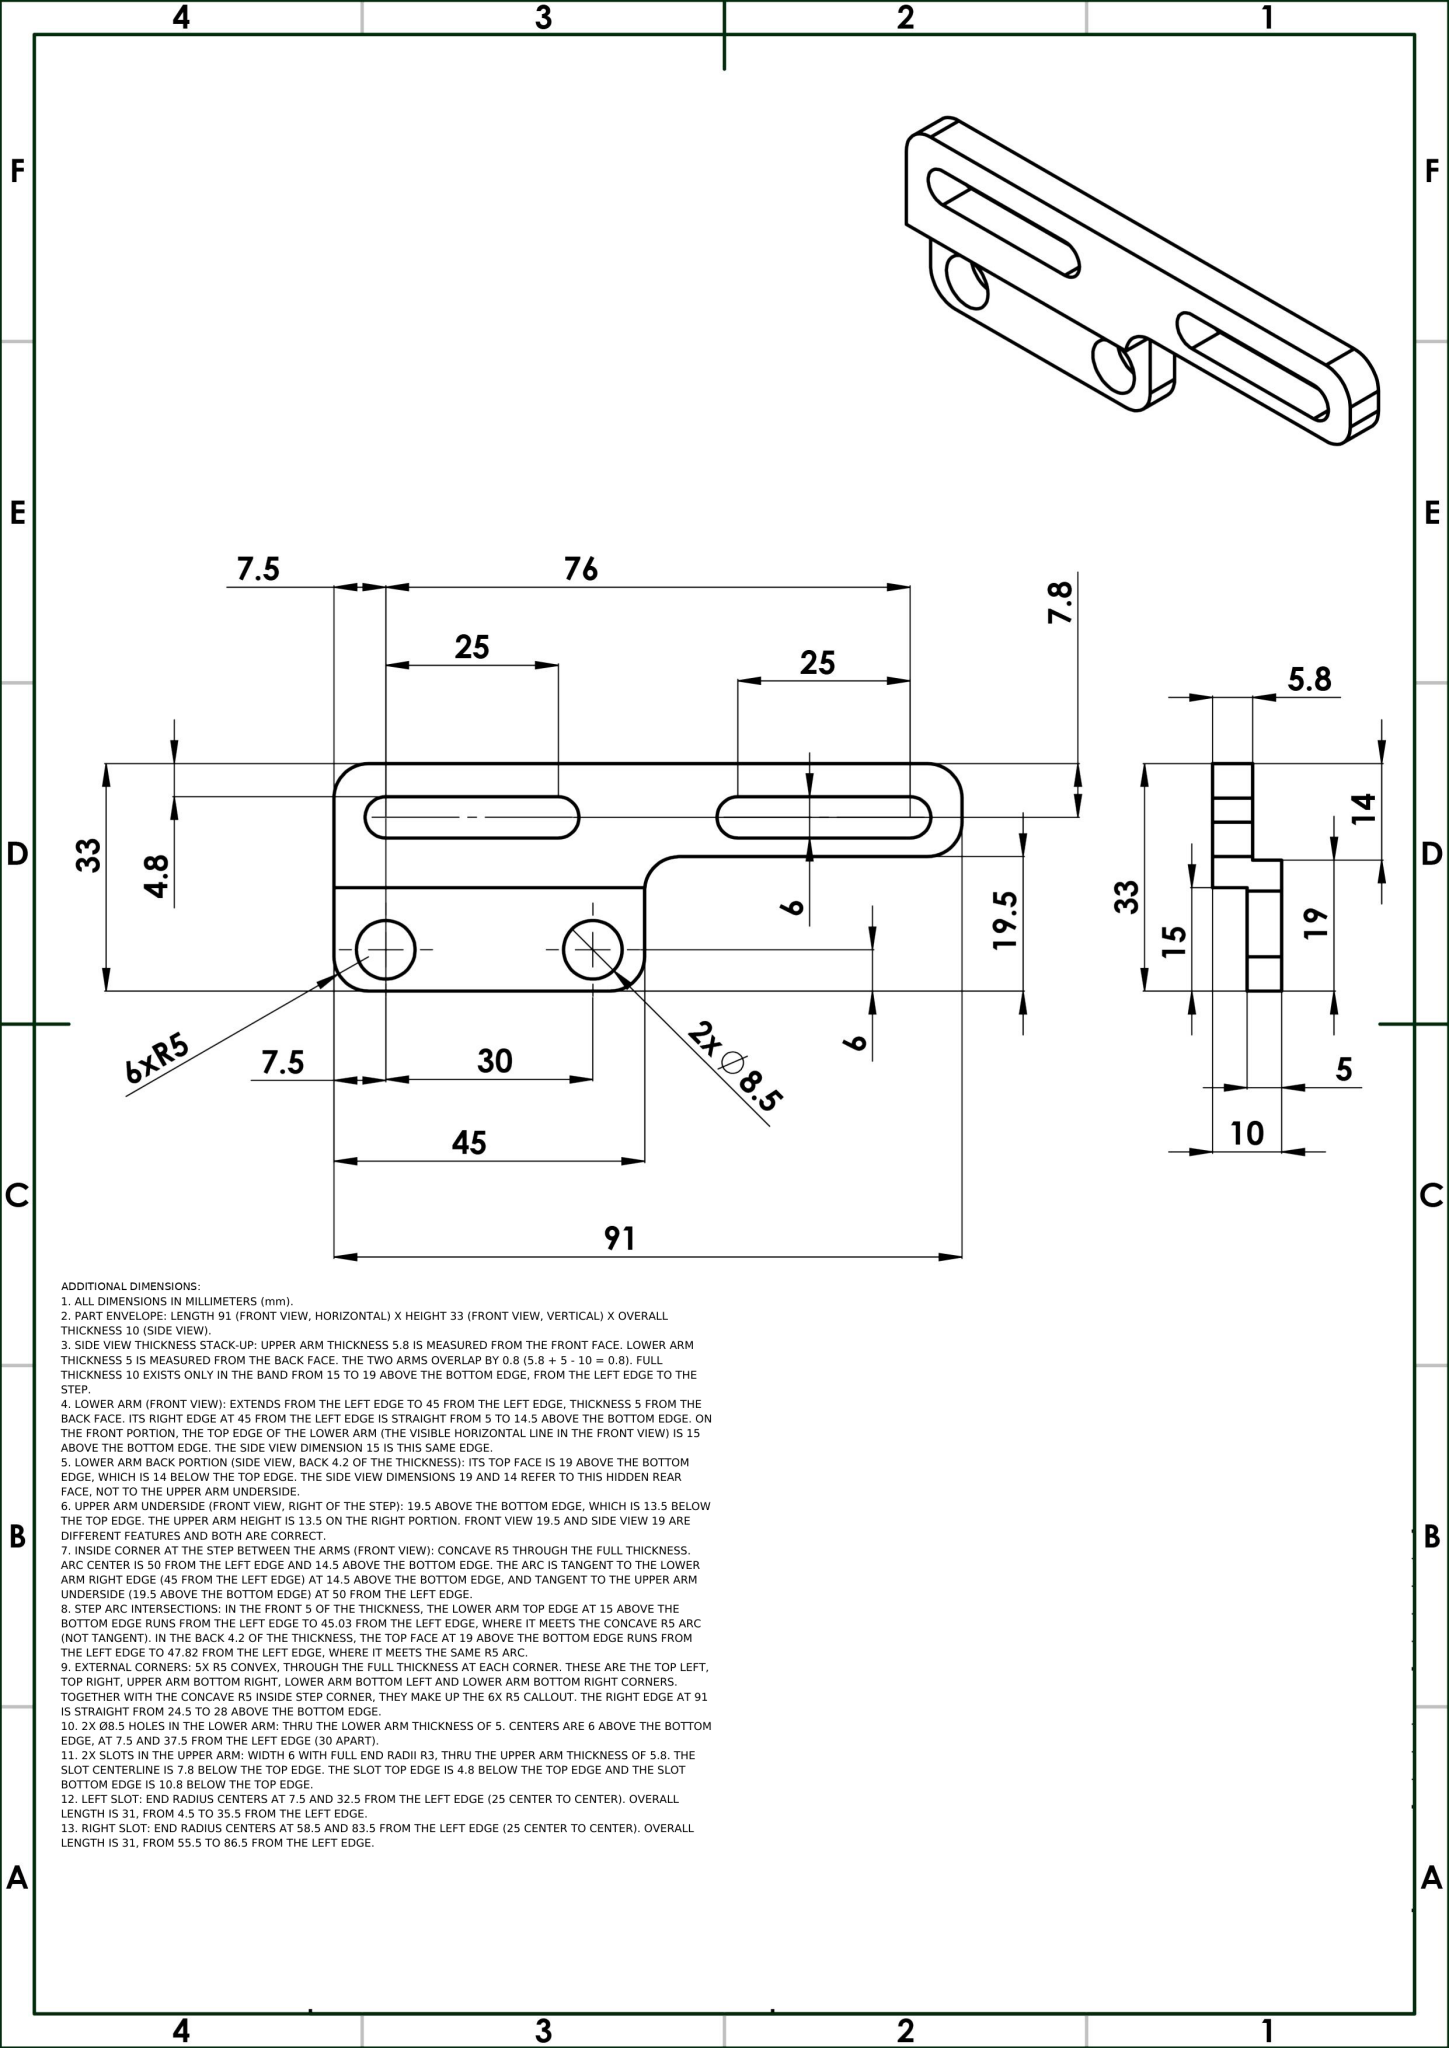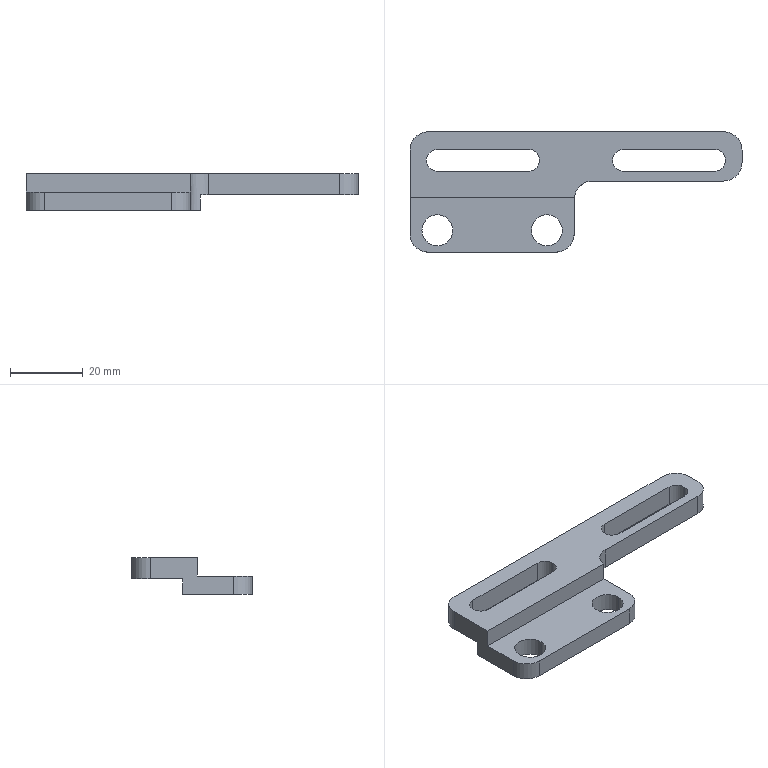Part | NX | mm | 1 solid | 32 faces | box 91 x 33 x 10 mm | volume 9695 mm3 | cylinder 16 | plane 16 | commonest cylinder face diameters 6 x6 10 x6 8.5 x4
STEP:
#1=CARTESIAN_POINT('',(11.75,-9.,0.));
#2=VERTEX_POINT('',#1);
#3=CARTESIAN_POINT('',(3.25,-9.,0.));
#4=VERTEX_POINT('',#3);
#5=CARTESIAN_POINT('',(7.5,-9.,0.));
#6=DIRECTION('',(0.,0.,-1.));
#7=DIRECTION('',(-1.,0.,0.));
#8=AXIS2_PLACEMENT_3D('',#5,#6,#7);
#9=CIRCLE('',#8,4.25);
#10=EDGE_CURVE('',#2,#4,#9,.T.);
#11=ORIENTED_EDGE('',*,*,#10,.F.);
#12=CARTESIAN_POINT('',(11.75,-9.,-5.));
#13=VERTEX_POINT('',#12);
#14=CARTESIAN_POINT('',(11.75,-9.,20.));
#15=DIRECTION('',(0.,0.,-1.));
#16=VECTOR('',#15,1000.);
#17=LINE('',#14,#16);
#18=EDGE_CURVE('',#2,#13,#17,.T.);
#19=ORIENTED_EDGE('',*,*,#18,.T.);
#20=CARTESIAN_POINT('',(3.25,-9.,-5.));
#21=VERTEX_POINT('',#20);
#22=CARTESIAN_POINT('',(7.5,-9.,-5.));
#23=DIRECTION('',(0.,0.,-1.));
#24=DIRECTION('',(-1.,0.,0.));
#25=AXIS2_PLACEMENT_3D('',#22,#23,#24);
#26=CIRCLE('',#25,4.25);
#27=EDGE_CURVE('',#13,#21,#26,.T.);
#28=ORIENTED_EDGE('',*,*,#27,.T.);
#29=CARTESIAN_POINT('',(3.25,-9.,20.));
#30=DIRECTION('',(0.,0.,-1.));
#31=VECTOR('',#30,1000.);
#32=LINE('',#29,#31);
#33=EDGE_CURVE('',#4,#21,#32,.T.);
#34=ORIENTED_EDGE('',*,*,#33,.F.);
#35=EDGE_LOOP('',(#11,#19,#28,#34));
#36=FACE_OUTER_BOUND('',#35,.T.);
#37=CARTESIAN_POINT('',(7.5,-9.,20.));
#38=DIRECTION('',(0.,0.,-1.));
#39=DIRECTION('',(-1.,0.,0.));
#40=AXIS2_PLACEMENT_3D('',#37,#38,#39);
#41=CYLINDRICAL_SURFACE('',#40,4.25);
#42=ADVANCED_FACE('',(#36),#41,.F.);
#43=CARTESIAN_POINT('',(41.75,-9.,0.));
#44=VERTEX_POINT('',#43);
#45=CARTESIAN_POINT('',(33.25,-9.,0.));
#46=VERTEX_POINT('',#45);
#47=CARTESIAN_POINT('',(37.5,-9.,0.));
#48=DIRECTION('',(0.,0.,-1.));
#49=DIRECTION('',(-1.,0.,0.));
#50=AXIS2_PLACEMENT_3D('',#47,#48,#49);
#51=CIRCLE('',#50,4.25);
#52=EDGE_CURVE('',#44,#46,#51,.T.);
#53=ORIENTED_EDGE('',*,*,#52,.F.);
#54=CARTESIAN_POINT('',(41.75,-9.,-5.));
#55=VERTEX_POINT('',#54);
#56=CARTESIAN_POINT('',(41.75,-9.,20.));
#57=DIRECTION('',(0.,0.,-1.));
#58=VECTOR('',#57,1000.);
#59=LINE('',#56,#58);
#60=EDGE_CURVE('',#44,#55,#59,.T.);
#61=ORIENTED_EDGE('',*,*,#60,.T.);
#62=CARTESIAN_POINT('',(33.25,-9.,-5.));
#63=VERTEX_POINT('',#62);
#64=CARTESIAN_POINT('',(37.5,-9.,-5.));
#65=DIRECTION('',(0.,0.,-1.));
#66=DIRECTION('',(-1.,0.,0.));
#67=AXIS2_PLACEMENT_3D('',#64,#65,#66);
#68=CIRCLE('',#67,4.25);
#69=EDGE_CURVE('',#55,#63,#68,.T.);
#70=ORIENTED_EDGE('',*,*,#69,.T.);
#71=CARTESIAN_POINT('',(33.25,-9.,20.));
#72=DIRECTION('',(0.,0.,-1.));
#73=VECTOR('',#72,1000.);
#74=LINE('',#71,#73);
#75=EDGE_CURVE('',#46,#63,#74,.T.);
#76=ORIENTED_EDGE('',*,*,#75,.F.);
#77=EDGE_LOOP('',(#53,#61,#70,#76));
#78=FACE_OUTER_BOUND('',#77,.T.);
#79=CARTESIAN_POINT('',(37.5,-9.,20.));
#80=DIRECTION('',(0.,0.,-1.));
#81=DIRECTION('',(-1.,0.,0.));
#82=AXIS2_PLACEMENT_3D('',#79,#80,#81);
#83=CYLINDRICAL_SURFACE('',#82,4.25);
#84=ADVANCED_FACE('',(#78),#83,.F.);
#85=CARTESIAN_POINT('',(83.5,13.2,-0.8));
#86=VERTEX_POINT('',#85);
#87=CARTESIAN_POINT('',(86.5,10.2,-0.8));
#88=VERTEX_POINT('',#87);
#89=CARTESIAN_POINT('',(83.5,10.2,-0.8));
#90=DIRECTION('',(0.,0.,-1.));
#91=DIRECTION('',(-1.,0.,0.));
#92=AXIS2_PLACEMENT_3D('',#89,#90,#91);
#93=CIRCLE('',#92,3.);
#94=EDGE_CURVE('',#86,#88,#93,.T.);
#95=ORIENTED_EDGE('',*,*,#94,.T.);
#96=CARTESIAN_POINT('',(86.5,10.2,5.));
#97=VERTEX_POINT('',#96);
#98=CARTESIAN_POINT('',(86.5,10.2,-5.));
#99=DIRECTION('',(0.,0.,1.));
#100=VECTOR('',#99,1000.);
#101=LINE('',#98,#100);
#102=EDGE_CURVE('',#88,#97,#101,.T.);
#103=ORIENTED_EDGE('',*,*,#102,.T.);
#104=CARTESIAN_POINT('',(83.5,13.2,5.));
#105=VERTEX_POINT('',#104);
#106=CARTESIAN_POINT('',(83.5,10.2,5.));
#107=DIRECTION('',(0.,0.,1.));
#108=DIRECTION('',(1.,0.,0.));
#109=AXIS2_PLACEMENT_3D('',#106,#107,#108);
#110=CIRCLE('',#109,3.);
#111=EDGE_CURVE('',#97,#105,#110,.T.);
#112=ORIENTED_EDGE('',*,*,#111,.T.);
#113=CARTESIAN_POINT('',(83.5,13.2,-5.));
#114=DIRECTION('',(0.,0.,1.));
#115=VECTOR('',#114,1000.);
#116=LINE('',#113,#115);
#117=EDGE_CURVE('',#86,#105,#116,.T.);
#118=ORIENTED_EDGE('',*,*,#117,.F.);
#119=EDGE_LOOP('',(#95,#103,#112,#118));
#120=FACE_OUTER_BOUND('',#119,.T.);
#121=CARTESIAN_POINT('',(83.5,10.2,-5.));
#122=DIRECTION('',(0.,0.,1.));
#123=DIRECTION('',(1.,0.,0.));
#124=AXIS2_PLACEMENT_3D('',#121,#122,#123);
#125=CYLINDRICAL_SURFACE('',#124,3.);
#126=ADVANCED_FACE('',(#120),#125,.F.);
#127=CARTESIAN_POINT('',(32.5,13.2,-0.8));
#128=VERTEX_POINT('',#127);
#129=CARTESIAN_POINT('',(35.5,10.2,-0.8));
#130=VERTEX_POINT('',#129);
#131=CARTESIAN_POINT('',(32.5,10.2,-0.8));
#132=DIRECTION('',(0.,0.,-1.));
#133=DIRECTION('',(-1.,0.,0.));
#134=AXIS2_PLACEMENT_3D('',#131,#132,#133);
#135=CIRCLE('',#134,3.);
#136=EDGE_CURVE('',#128,#130,#135,.T.);
#137=ORIENTED_EDGE('',*,*,#136,.T.);
#138=CARTESIAN_POINT('',(35.5,10.2,5.));
#139=VERTEX_POINT('',#138);
#140=CARTESIAN_POINT('',(35.5,10.2,-5.));
#141=DIRECTION('',(0.,0.,1.));
#142=VECTOR('',#141,1000.);
#143=LINE('',#140,#142);
#144=EDGE_CURVE('',#130,#139,#143,.T.);
#145=ORIENTED_EDGE('',*,*,#144,.T.);
#146=CARTESIAN_POINT('',(32.5,13.2,5.));
#147=VERTEX_POINT('',#146);
#148=CARTESIAN_POINT('',(32.5,10.2,5.));
#149=DIRECTION('',(0.,0.,1.));
#150=DIRECTION('',(1.,0.,0.));
#151=AXIS2_PLACEMENT_3D('',#148,#149,#150);
#152=CIRCLE('',#151,3.);
#153=EDGE_CURVE('',#139,#147,#152,.T.);
#154=ORIENTED_EDGE('',*,*,#153,.T.);
#155=CARTESIAN_POINT('',(32.5,13.2,-5.));
#156=DIRECTION('',(0.,0.,1.));
#157=VECTOR('',#156,1000.);
#158=LINE('',#155,#157);
#159=EDGE_CURVE('',#128,#147,#158,.T.);
#160=ORIENTED_EDGE('',*,*,#159,.F.);
#161=EDGE_LOOP('',(#137,#145,#154,#160));
#162=FACE_OUTER_BOUND('',#161,.T.);
#163=CARTESIAN_POINT('',(32.5,10.2,-5.));
#164=DIRECTION('',(0.,0.,1.));
#165=DIRECTION('',(1.,0.,0.));
#166=AXIS2_PLACEMENT_3D('',#163,#164,#165);
#167=CYLINDRICAL_SURFACE('',#166,3.);
#168=ADVANCED_FACE('',(#162),#167,.F.);
#169=CARTESIAN_POINT('',(45.025,0.,0.));
#170=VERTEX_POINT('',#169);
#171=CARTESIAN_POINT('',(0.,0.,0.));
#172=VERTEX_POINT('',#171);
#173=CARTESIAN_POINT('',(0.,0.,0.));
#174=DIRECTION('',(-1.,0.,0.));
#175=VECTOR('',#174,1000.);
#176=LINE('',#173,#175);
#177=EDGE_CURVE('',#170,#172,#176,.T.);
#178=ORIENTED_EDGE('',*,*,#177,.F.);
#179=CARTESIAN_POINT('',(45.025,0.,5.));
#180=VERTEX_POINT('',#179);
#181=CARTESIAN_POINT('',(45.025,0.,0.));
#182=DIRECTION('',(0.,0.,1.));
#183=VECTOR('',#182,1000.);
#184=LINE('',#181,#183);
#185=EDGE_CURVE('',#170,#180,#184,.T.);
#186=ORIENTED_EDGE('',*,*,#185,.T.);
#187=CARTESIAN_POINT('',(0.,0.,5.));
#188=VERTEX_POINT('',#187);
#189=CARTESIAN_POINT('',(0.,0.,5.));
#190=DIRECTION('',(1.,0.,0.));
#191=VECTOR('',#190,1000.);
#192=LINE('',#189,#191);
#193=EDGE_CURVE('',#188,#180,#192,.T.);
#194=ORIENTED_EDGE('',*,*,#193,.F.);
#195=CARTESIAN_POINT('',(0.,0.,5.));
#196=DIRECTION('',(0.,0.,-1.));
#197=VECTOR('',#196,1000.);
#198=LINE('',#195,#197);
#199=EDGE_CURVE('',#188,#172,#198,.T.);
#200=ORIENTED_EDGE('',*,*,#199,.T.);
#201=EDGE_LOOP('',(#178,#186,#194,#200));
#202=FACE_OUTER_BOUND('',#201,.T.);
#203=CARTESIAN_POINT('',(0.,0.,5.));
#204=DIRECTION('',(0.,1.,0.));
#205=DIRECTION('',(0.,0.,1.));
#206=AXIS2_PLACEMENT_3D('',#203,#204,#205);
#207=PLANE('',#206);
#208=ADVANCED_FACE('',(#202),#207,.F.);
#209=CARTESIAN_POINT('',(0.,-10.,-5.));
#210=VERTEX_POINT('',#209);
#211=CARTESIAN_POINT('',(0.,4.,-5.));
#212=VERTEX_POINT('',#211);
#213=CARTESIAN_POINT('',(0.,0.,-5.));
#214=DIRECTION('',(0.,1.,0.));
#215=VECTOR('',#214,1000.);
#216=LINE('',#213,#215);
#217=EDGE_CURVE('',#210,#212,#216,.T.);
#218=ORIENTED_EDGE('',*,*,#217,.F.);
#219=CARTESIAN_POINT('',(0.,-10.,0.));
#220=VERTEX_POINT('',#219);
#221=CARTESIAN_POINT('',(0.,-10.,5.));
#222=DIRECTION('',(0.,0.,1.));
#223=VECTOR('',#222,1000.);
#224=LINE('',#221,#223);
#225=EDGE_CURVE('',#210,#220,#224,.T.);
#226=ORIENTED_EDGE('',*,*,#225,.T.);
#227=CARTESIAN_POINT('',(0.,-15.,0.));
#228=DIRECTION('',(0.,1.,0.));
#229=VECTOR('',#228,1000.);
#230=LINE('',#227,#229);
#231=EDGE_CURVE('',#220,#172,#230,.T.);
#232=ORIENTED_EDGE('',*,*,#231,.T.);
#233=ORIENTED_EDGE('',*,*,#199,.F.);
#234=CARTESIAN_POINT('',(0.,13.,5.));
#235=VERTEX_POINT('',#234);
#236=CARTESIAN_POINT('',(0.,0.,5.));
#237=DIRECTION('',(0.,-1.,0.));
#238=VECTOR('',#237,1000.);
#239=LINE('',#236,#238);
#240=EDGE_CURVE('',#235,#188,#239,.T.);
#241=ORIENTED_EDGE('',*,*,#240,.F.);
#242=CARTESIAN_POINT('',(0.,13.,-0.8));
#243=VERTEX_POINT('',#242);
#244=CARTESIAN_POINT('',(0.,13.,5.));
#245=DIRECTION('',(0.,0.,-1.));
#246=VECTOR('',#245,1000.);
#247=LINE('',#244,#246);
#248=EDGE_CURVE('',#235,#243,#247,.T.);
#249=ORIENTED_EDGE('',*,*,#248,.T.);
#250=CARTESIAN_POINT('',(0.,4.,-0.8));
#251=VERTEX_POINT('',#250);
#252=CARTESIAN_POINT('',(0.,4.,-0.8));
#253=DIRECTION('',(0.,1.,0.));
#254=VECTOR('',#253,1000.);
#255=LINE('',#252,#254);
#256=EDGE_CURVE('',#251,#243,#255,.T.);
#257=ORIENTED_EDGE('',*,*,#256,.F.);
#258=CARTESIAN_POINT('',(0.,4.,-5.));
#259=DIRECTION('',(0.,0.,1.));
#260=VECTOR('',#259,1000.);
#261=LINE('',#258,#260);
#262=EDGE_CURVE('',#212,#251,#261,.T.);
#263=ORIENTED_EDGE('',*,*,#262,.F.);
#264=EDGE_LOOP('',(#218,#226,#232,#233,#241,#249,#257,#263));
#265=FACE_OUTER_BOUND('',#264,.T.);
#266=CARTESIAN_POINT('',(0.,0.,5.));
#267=DIRECTION('',(1.,0.,0.));
#268=DIRECTION('',(0.,0.,-1.));
#269=AXIS2_PLACEMENT_3D('',#266,#267,#268);
#270=PLANE('',#269);
#271=ADVANCED_FACE('',(#265),#270,.F.);
#272=CARTESIAN_POINT('',(91.,9.5,5.));
#273=VERTEX_POINT('',#272);
#274=CARTESIAN_POINT('',(91.,13.,5.));
#275=VERTEX_POINT('',#274);
#276=CARTESIAN_POINT('',(91.,0.,5.));
#277=DIRECTION('',(0.,1.,0.));
#278=VECTOR('',#277,1000.);
#279=LINE('',#276,#278);
#280=EDGE_CURVE('',#273,#275,#279,.T.);
#281=ORIENTED_EDGE('',*,*,#280,.F.);
#282=CARTESIAN_POINT('',(91.,9.5,-0.8));
#283=VERTEX_POINT('',#282);
#284=CARTESIAN_POINT('',(91.,9.5,5.));
#285=DIRECTION('',(0.,0.,-1.));
#286=VECTOR('',#285,1000.);
#287=LINE('',#284,#286);
#288=EDGE_CURVE('',#273,#283,#287,.T.);
#289=ORIENTED_EDGE('',*,*,#288,.T.);
#290=CARTESIAN_POINT('',(91.,13.,-0.8));
#291=VERTEX_POINT('',#290);
#292=CARTESIAN_POINT('',(91.,18.,-0.8));
#293=DIRECTION('',(0.,-1.,0.));
#294=VECTOR('',#293,1000.);
#295=LINE('',#292,#294);
#296=EDGE_CURVE('',#291,#283,#295,.T.);
#297=ORIENTED_EDGE('',*,*,#296,.F.);
#298=CARTESIAN_POINT('',(91.,13.,5.));
#299=DIRECTION('',(0.,0.,1.));
#300=VECTOR('',#299,1000.);
#301=LINE('',#298,#300);
#302=EDGE_CURVE('',#291,#275,#301,.T.);
#303=ORIENTED_EDGE('',*,*,#302,.T.);
#304=EDGE_LOOP('',(#281,#289,#297,#303));
#305=FACE_OUTER_BOUND('',#304,.T.);
#306=CARTESIAN_POINT('',(91.,0.,5.));
#307=DIRECTION('',(-1.,0.,0.));
#308=DIRECTION('',(0.,0.,1.));
#309=AXIS2_PLACEMENT_3D('',#306,#307,#308);
#310=PLANE('',#309);
#311=ADVANCED_FACE('',(#305),#310,.F.);
#312=CARTESIAN_POINT('',(5.,18.,-0.8));
#313=VERTEX_POINT('',#312);
#314=CARTESIAN_POINT('',(86.,18.,-0.8));
#315=VERTEX_POINT('',#314);
#316=CARTESIAN_POINT('',(0.,18.,-0.8));
#317=DIRECTION('',(1.,0.,0.));
#318=VECTOR('',#317,1000.);
#319=LINE('',#316,#318);
#320=EDGE_CURVE('',#313,#315,#319,.T.);
#321=ORIENTED_EDGE('',*,*,#320,.F.);
#322=CARTESIAN_POINT('',(5.,18.,5.));
#323=VERTEX_POINT('',#322);
#324=CARTESIAN_POINT('',(5.,18.,5.));
#325=DIRECTION('',(0.,0.,1.));
#326=VECTOR('',#325,1000.);
#327=LINE('',#324,#326);
#328=EDGE_CURVE('',#313,#323,#327,.T.);
#329=ORIENTED_EDGE('',*,*,#328,.T.);
#330=CARTESIAN_POINT('',(86.,18.,5.));
#331=VERTEX_POINT('',#330);
#332=CARTESIAN_POINT('',(0.,18.,5.));
#333=DIRECTION('',(-1.,0.,0.));
#334=VECTOR('',#333,1000.);
#335=LINE('',#332,#334);
#336=EDGE_CURVE('',#331,#323,#335,.T.);
#337=ORIENTED_EDGE('',*,*,#336,.F.);
#338=CARTESIAN_POINT('',(86.,18.,5.));
#339=DIRECTION('',(0.,0.,-1.));
#340=VECTOR('',#339,1000.);
#341=LINE('',#338,#340);
#342=EDGE_CURVE('',#331,#315,#341,.T.);
#343=ORIENTED_EDGE('',*,*,#342,.T.);
#344=EDGE_LOOP('',(#321,#329,#337,#343));
#345=FACE_OUTER_BOUND('',#344,.T.);
#346=CARTESIAN_POINT('',(0.,18.,5.));
#347=DIRECTION('',(0.,-1.,0.));
#348=DIRECTION('',(0.,0.,-1.));
#349=AXIS2_PLACEMENT_3D('',#346,#347,#348);
#350=PLANE('',#349);
#351=ADVANCED_FACE('',(#345),#350,.F.);
#352=CARTESIAN_POINT('',(58.5,7.2,5.));
#353=VERTEX_POINT('',#352);
#354=CARTESIAN_POINT('',(83.5,7.2,5.));
#355=VERTEX_POINT('',#354);
#356=CARTESIAN_POINT('',(58.5,7.2,5.));
#357=DIRECTION('',(1.,0.,0.));
#358=VECTOR('',#357,1000.);
#359=LINE('',#356,#358);
#360=EDGE_CURVE('',#353,#355,#359,.T.);
#361=ORIENTED_EDGE('',*,*,#360,.F.);
#362=CARTESIAN_POINT('',(58.5,13.2,5.));
#363=VERTEX_POINT('',#362);
#364=CARTESIAN_POINT('',(58.5,10.2,5.));
#365=DIRECTION('',(0.,0.,1.));
#366=DIRECTION('',(1.,0.,0.));
#367=AXIS2_PLACEMENT_3D('',#364,#365,#366);
#368=CIRCLE('',#367,3.);
#369=EDGE_CURVE('',#363,#353,#368,.T.);
#370=ORIENTED_EDGE('',*,*,#369,.F.);
#371=CARTESIAN_POINT('',(58.5,13.2,5.));
#372=DIRECTION('',(-1.,-0.,0.));
#373=VECTOR('',#372,1000.);
#374=LINE('',#371,#373);
#375=EDGE_CURVE('',#105,#363,#374,.T.);
#376=ORIENTED_EDGE('',*,*,#375,.F.);
#377=ORIENTED_EDGE('',*,*,#111,.F.);
#378=CARTESIAN_POINT('',(83.5,10.2,5.));
#379=DIRECTION('',(0.,0.,1.));
#380=DIRECTION('',(1.,0.,0.));
#381=AXIS2_PLACEMENT_3D('',#378,#379,#380);
#382=CIRCLE('',#381,3.);
#383=EDGE_CURVE('',#355,#97,#382,.T.);
#384=ORIENTED_EDGE('',*,*,#383,.F.);
#385=EDGE_LOOP('',(#361,#370,#376,#377,#384));
#386=FACE_BOUND('',#385,.T.);
#387=CARTESIAN_POINT('',(7.5,7.2,5.));
#388=VERTEX_POINT('',#387);
#389=CARTESIAN_POINT('',(32.5,7.2,5.));
#390=VERTEX_POINT('',#389);
#391=CARTESIAN_POINT('',(7.5,7.2,5.));
#392=DIRECTION('',(1.,0.,0.));
#393=VECTOR('',#392,1000.);
#394=LINE('',#391,#393);
#395=EDGE_CURVE('',#388,#390,#394,.T.);
#396=ORIENTED_EDGE('',*,*,#395,.F.);
#397=CARTESIAN_POINT('',(7.5,13.2,5.));
#398=VERTEX_POINT('',#397);
#399=CARTESIAN_POINT('',(7.5,10.2,5.));
#400=DIRECTION('',(0.,0.,1.));
#401=DIRECTION('',(1.,0.,0.));
#402=AXIS2_PLACEMENT_3D('',#399,#400,#401);
#403=CIRCLE('',#402,3.);
#404=EDGE_CURVE('',#398,#388,#403,.T.);
#405=ORIENTED_EDGE('',*,*,#404,.F.);
#406=CARTESIAN_POINT('',(7.5,13.2,5.));
#407=DIRECTION('',(-1.,-0.,0.));
#408=VECTOR('',#407,1000.);
#409=LINE('',#406,#408);
#410=EDGE_CURVE('',#147,#398,#409,.T.);
#411=ORIENTED_EDGE('',*,*,#410,.F.);
#412=ORIENTED_EDGE('',*,*,#153,.F.);
#413=CARTESIAN_POINT('',(32.5,10.2,5.));
#414=DIRECTION('',(0.,0.,1.));
#415=DIRECTION('',(1.,0.,0.));
#416=AXIS2_PLACEMENT_3D('',#413,#414,#415);
#417=CIRCLE('',#416,3.);
#418=EDGE_CURVE('',#390,#139,#417,.T.);
#419=ORIENTED_EDGE('',*,*,#418,.F.);
#420=EDGE_LOOP('',(#396,#405,#411,#412,#419));
#421=FACE_BOUND('',#420,.T.);
#422=CARTESIAN_POINT('',(50.,4.5,5.));
#423=VERTEX_POINT('',#422);
#424=CARTESIAN_POINT('',(86.,4.5,5.));
#425=VERTEX_POINT('',#424);
#426=CARTESIAN_POINT('',(0.,4.5,5.));
#427=DIRECTION('',(1.,0.,0.));
#428=VECTOR('',#427,1000.);
#429=LINE('',#426,#428);
#430=EDGE_CURVE('',#423,#425,#429,.T.);
#431=ORIENTED_EDGE('',*,*,#430,.T.);
#432=CARTESIAN_POINT('',(86.,9.5,5.));
#433=DIRECTION('',(0.,0.,1.));
#434=DIRECTION('',(-1.,0.,0.));
#435=AXIS2_PLACEMENT_3D('',#432,#433,#434);
#436=CIRCLE('',#435,5.);
#437=EDGE_CURVE('',#425,#273,#436,.T.);
#438=ORIENTED_EDGE('',*,*,#437,.T.);
#439=ORIENTED_EDGE('',*,*,#280,.T.);
#440=CARTESIAN_POINT('',(86.,13.,5.));
#441=DIRECTION('',(0.,0.,1.));
#442=DIRECTION('',(-1.,0.,0.));
#443=AXIS2_PLACEMENT_3D('',#440,#441,#442);
#444=CIRCLE('',#443,5.);
#445=EDGE_CURVE('',#275,#331,#444,.T.);
#446=ORIENTED_EDGE('',*,*,#445,.T.);
#447=ORIENTED_EDGE('',*,*,#336,.T.);
#448=CARTESIAN_POINT('',(5.,13.,5.));
#449=DIRECTION('',(0.,0.,1.));
#450=DIRECTION('',(-1.,0.,0.));
#451=AXIS2_PLACEMENT_3D('',#448,#449,#450);
#452=CIRCLE('',#451,5.);
#453=EDGE_CURVE('',#323,#235,#452,.T.);
#454=ORIENTED_EDGE('',*,*,#453,.T.);
#455=ORIENTED_EDGE('',*,*,#240,.T.);
#456=ORIENTED_EDGE('',*,*,#193,.T.);
#457=CARTESIAN_POINT('',(50.,-0.5,5.));
#458=DIRECTION('',(0.,0.,-1.));
#459=DIRECTION('',(-1.,0.,0.));
#460=AXIS2_PLACEMENT_3D('',#457,#458,#459);
#461=CIRCLE('',#460,5.);
#462=EDGE_CURVE('',#180,#423,#461,.T.);
#463=ORIENTED_EDGE('',*,*,#462,.T.);
#464=EDGE_LOOP('',(#431,#438,#439,#446,#447,#454,#455,#456,#463));
#465=FACE_OUTER_BOUND('',#464,.T.);
#466=CARTESIAN_POINT('',(0.,0.,5.));
#467=DIRECTION('',(0.,0.,-1.));
#468=DIRECTION('',(-1.,0.,0.));
#469=AXIS2_PLACEMENT_3D('',#466,#467,#468);
#470=PLANE('',#469);
#471=ADVANCED_FACE('',(#386,#421,#465),#470,.F.);
#472=CARTESIAN_POINT('',(7.5,7.2,-0.8));
#473=VERTEX_POINT('',#472);
#474=CARTESIAN_POINT('',(7.5,7.2,-5.));
#475=DIRECTION('',(0.,0.,1.));
#476=VECTOR('',#475,1000.);
#477=LINE('',#474,#476);
#478=EDGE_CURVE('',#473,#388,#477,.T.);
#479=ORIENTED_EDGE('',*,*,#478,.F.);
#480=CARTESIAN_POINT('',(7.5,13.2,-0.8));
#481=VERTEX_POINT('',#480);
#482=CARTESIAN_POINT('',(7.5,10.2,-0.8));
#483=DIRECTION('',(0.,0.,-1.));
#484=DIRECTION('',(-1.,0.,0.));
#485=AXIS2_PLACEMENT_3D('',#482,#483,#484);
#486=CIRCLE('',#485,3.);
#487=EDGE_CURVE('',#473,#481,#486,.T.);
#488=ORIENTED_EDGE('',*,*,#487,.T.);
#489=CARTESIAN_POINT('',(7.5,13.2,-5.));
#490=DIRECTION('',(0.,0.,1.));
#491=VECTOR('',#490,1000.);
#492=LINE('',#489,#491);
#493=EDGE_CURVE('',#481,#398,#492,.T.);
#494=ORIENTED_EDGE('',*,*,#493,.T.);
#495=ORIENTED_EDGE('',*,*,#404,.T.);
#496=EDGE_LOOP('',(#479,#488,#494,#495));
#497=FACE_OUTER_BOUND('',#496,.T.);
#498=CARTESIAN_POINT('',(7.5,10.2,-5.));
#499=DIRECTION('',(0.,0.,1.));
#500=DIRECTION('',(1.,0.,0.));
#501=AXIS2_PLACEMENT_3D('',#498,#499,#500);
#502=CYLINDRICAL_SURFACE('',#501,3.);
#503=ADVANCED_FACE('',(#497),#502,.F.);
#504=ORIENTED_EDGE('',*,*,#493,.F.);
#505=CARTESIAN_POINT('',(32.5,13.2,-0.8));
#506=DIRECTION('',(1.,0.,0.));
#507=VECTOR('',#506,1000.);
#508=LINE('',#505,#507);
#509=EDGE_CURVE('',#481,#128,#508,.T.);
#510=ORIENTED_EDGE('',*,*,#509,.T.);
#511=ORIENTED_EDGE('',*,*,#159,.T.);
#512=ORIENTED_EDGE('',*,*,#410,.T.);
#513=EDGE_LOOP('',(#504,#510,#511,#512));
#514=FACE_OUTER_BOUND('',#513,.T.);
#515=CARTESIAN_POINT('',(7.5,13.2,-5.));
#516=DIRECTION('',(-0.,1.,0.));
#517=DIRECTION('',(-1.,-0.,0.));
#518=AXIS2_PLACEMENT_3D('',#515,#516,#517);
#519=PLANE('',#518);
#520=ADVANCED_FACE('',(#514),#519,.F.);
#521=ORIENTED_EDGE('',*,*,#144,.F.);
#522=CARTESIAN_POINT('',(32.5,7.2,-0.8));
#523=VERTEX_POINT('',#522);
#524=CARTESIAN_POINT('',(32.5,10.2,-0.8));
#525=DIRECTION('',(0.,0.,-1.));
#526=DIRECTION('',(-1.,0.,0.));
#527=AXIS2_PLACEMENT_3D('',#524,#525,#526);
#528=CIRCLE('',#527,3.);
#529=EDGE_CURVE('',#130,#523,#528,.T.);
#530=ORIENTED_EDGE('',*,*,#529,.T.);
#531=CARTESIAN_POINT('',(32.5,7.2,-5.));
#532=DIRECTION('',(0.,0.,1.));
#533=VECTOR('',#532,1000.);
#534=LINE('',#531,#533);
#535=EDGE_CURVE('',#523,#390,#534,.T.);
#536=ORIENTED_EDGE('',*,*,#535,.T.);
#537=ORIENTED_EDGE('',*,*,#418,.T.);
#538=EDGE_LOOP('',(#521,#530,#536,#537));
#539=FACE_OUTER_BOUND('',#538,.T.);
#540=CARTESIAN_POINT('',(32.5,10.2,-5.));
#541=DIRECTION('',(0.,0.,1.));
#542=DIRECTION('',(1.,0.,0.));
#543=AXIS2_PLACEMENT_3D('',#540,#541,#542);
#544=CYLINDRICAL_SURFACE('',#543,3.);
#545=ADVANCED_FACE('',(#539),#544,.F.);
#546=ORIENTED_EDGE('',*,*,#535,.F.);
#547=CARTESIAN_POINT('',(32.5,7.2,-0.8));
#548=DIRECTION('',(-1.,0.,0.));
#549=VECTOR('',#548,1000.);
#550=LINE('',#547,#549);
#551=EDGE_CURVE('',#523,#473,#550,.T.);
#552=ORIENTED_EDGE('',*,*,#551,.T.);
#553=ORIENTED_EDGE('',*,*,#478,.T.);
#554=ORIENTED_EDGE('',*,*,#395,.T.);
#555=EDGE_LOOP('',(#546,#552,#553,#554));
#556=FACE_OUTER_BOUND('',#555,.T.);
#557=CARTESIAN_POINT('',(7.5,7.2,-5.));
#558=DIRECTION('',(0.,-1.,0.));
#559=DIRECTION('',(1.,0.,0.));
#560=AXIS2_PLACEMENT_3D('',#557,#558,#559);
#561=PLANE('',#560);
#562=ADVANCED_FACE('',(#556),#561,.F.);
#563=CARTESIAN_POINT('',(58.5,7.2,-0.8));
#564=VERTEX_POINT('',#563);
#565=CARTESIAN_POINT('',(58.5,7.2,-5.));
#566=DIRECTION('',(0.,0.,1.));
#567=VECTOR('',#566,1000.);
#568=LINE('',#565,#567);
#569=EDGE_CURVE('',#564,#353,#568,.T.);
#570=ORIENTED_EDGE('',*,*,#569,.F.);
#571=CARTESIAN_POINT('',(58.5,13.2,-0.8));
#572=VERTEX_POINT('',#571);
#573=CARTESIAN_POINT('',(58.5,10.2,-0.8));
#574=DIRECTION('',(0.,0.,-1.));
#575=DIRECTION('',(-1.,0.,0.));
#576=AXIS2_PLACEMENT_3D('',#573,#574,#575);
#577=CIRCLE('',#576,3.);
#578=EDGE_CURVE('',#564,#572,#577,.T.);
#579=ORIENTED_EDGE('',*,*,#578,.T.);
#580=CARTESIAN_POINT('',(58.5,13.2,-5.));
#581=DIRECTION('',(0.,0.,1.));
#582=VECTOR('',#581,1000.);
#583=LINE('',#580,#582);
#584=EDGE_CURVE('',#572,#363,#583,.T.);
#585=ORIENTED_EDGE('',*,*,#584,.T.);
#586=ORIENTED_EDGE('',*,*,#369,.T.);
#587=EDGE_LOOP('',(#570,#579,#585,#586));
#588=FACE_OUTER_BOUND('',#587,.T.);
#589=CARTESIAN_POINT('',(58.5,10.2,-5.));
#590=DIRECTION('',(0.,0.,1.));
#591=DIRECTION('',(1.,0.,0.));
#592=AXIS2_PLACEMENT_3D('',#589,#590,#591);
#593=CYLINDRICAL_SURFACE('',#592,3.);
#594=ADVANCED_FACE('',(#588),#593,.F.);
#595=ORIENTED_EDGE('',*,*,#584,.F.);
#596=CARTESIAN_POINT('',(83.5,13.2,-0.8));
#597=DIRECTION('',(1.,-0.,0.));
#598=VECTOR('',#597,1000.);
#599=LINE('',#596,#598);
#600=EDGE_CURVE('',#572,#86,#599,.T.);
#601=ORIENTED_EDGE('',*,*,#600,.T.);
#602=ORIENTED_EDGE('',*,*,#117,.T.);
#603=ORIENTED_EDGE('',*,*,#375,.T.);
#604=EDGE_LOOP('',(#595,#601,#602,#603));
#605=FACE_OUTER_BOUND('',#604,.T.);
#606=CARTESIAN_POINT('',(58.5,13.2,-5.));
#607=DIRECTION('',(-0.,1.,0.));
#608=DIRECTION('',(-1.,-0.,0.));
#609=AXIS2_PLACEMENT_3D('',#606,#607,#608);
#610=PLANE('',#609);
#611=ADVANCED_FACE('',(#605),#610,.F.);
#612=ORIENTED_EDGE('',*,*,#102,.F.);
#613=CARTESIAN_POINT('',(83.5,7.2,-0.8));
#614=VERTEX_POINT('',#613);
#615=CARTESIAN_POINT('',(83.5,10.2,-0.8));
#616=DIRECTION('',(0.,0.,-1.));
#617=DIRECTION('',(-1.,0.,0.));
#618=AXIS2_PLACEMENT_3D('',#615,#616,#617);
#619=CIRCLE('',#618,3.);
#620=EDGE_CURVE('',#88,#614,#619,.T.);
#621=ORIENTED_EDGE('',*,*,#620,.T.);
#622=CARTESIAN_POINT('',(83.5,7.2,-5.));
#623=DIRECTION('',(0.,0.,1.));
#624=VECTOR('',#623,1000.);
#625=LINE('',#622,#624);
#626=EDGE_CURVE('',#614,#355,#625,.T.);
#627=ORIENTED_EDGE('',*,*,#626,.T.);
#628=ORIENTED_EDGE('',*,*,#383,.T.);
#629=EDGE_LOOP('',(#612,#621,#627,#628));
#630=FACE_OUTER_BOUND('',#629,.T.);
#631=CARTESIAN_POINT('',(83.5,10.2,-5.));
#632=DIRECTION('',(0.,0.,1.));
#633=DIRECTION('',(1.,0.,0.));
#634=AXIS2_PLACEMENT_3D('',#631,#632,#633);
#635=CYLINDRICAL_SURFACE('',#634,3.);
#636=ADVANCED_FACE('',(#630),#635,.F.);
#637=ORIENTED_EDGE('',*,*,#626,.F.);
#638=CARTESIAN_POINT('',(83.5,7.2,-0.8));
#639=DIRECTION('',(-1.,-0.,0.));
#640=VECTOR('',#639,1000.);
#641=LINE('',#638,#640);
#642=EDGE_CURVE('',#614,#564,#641,.T.);
#643=ORIENTED_EDGE('',*,*,#642,.T.);
#644=ORIENTED_EDGE('',*,*,#569,.T.);
#645=ORIENTED_EDGE('',*,*,#360,.T.);
#646=EDGE_LOOP('',(#637,#643,#644,#645));
#647=FACE_OUTER_BOUND('',#646,.T.);
#648=CARTESIAN_POINT('',(58.5,7.2,-5.));
#649=DIRECTION('',(0.,-1.,0.));
#650=DIRECTION('',(1.,0.,0.));
#651=AXIS2_PLACEMENT_3D('',#648,#649,#650);
#652=PLANE('',#651);
#653=ADVANCED_FACE('',(#647),#652,.F.);
#654=ORIENTED_EDGE('',*,*,#262,.T.);
#655=CARTESIAN_POINT('',(47.821,4.,-0.8));
#656=VERTEX_POINT('',#655);
#657=CARTESIAN_POINT('',(91.,4.,-0.8));
#658=DIRECTION('',(-1.,0.,0.));
#659=VECTOR('',#658,1000.);
#660=LINE('',#657,#659);
#661=EDGE_CURVE('',#656,#251,#660,.T.);
#662=ORIENTED_EDGE('',*,*,#661,.F.);
#663=CARTESIAN_POINT('',(47.821,4.,-5.));
#664=VERTEX_POINT('',#663);
#665=CARTESIAN_POINT('',(47.821,4.,-0.8));
#666=DIRECTION('',(0.,0.,-1.));
#667=VECTOR('',#666,1000.);
#668=LINE('',#665,#667);
#669=EDGE_CURVE('',#656,#664,#668,.T.);
#670=ORIENTED_EDGE('',*,*,#669,.T.);
#671=CARTESIAN_POINT('',(0.,4.,-5.));
#672=DIRECTION('',(1.,-0.,0.));
#673=VECTOR('',#672,1000.);
#674=LINE('',#671,#673);
#675=EDGE_CURVE('',#212,#664,#674,.T.);
#676=ORIENTED_EDGE('',*,*,#675,.F.);
#677=EDGE_LOOP('',(#654,#662,#670,#676));
#678=FACE_OUTER_BOUND('',#677,.T.);
#679=CARTESIAN_POINT('',(0.,4.,-5.));
#680=DIRECTION('',(-0.,-1.,0.));
#681=DIRECTION('',(1.,-0.,0.));
#682=AXIS2_PLACEMENT_3D('',#679,#680,#681);
#683=PLANE('',#682);
#684=ADVANCED_FACE('',(#678),#683,.F.);
#685=CARTESIAN_POINT('',(45.,-10.,0.));
#686=VERTEX_POINT('',#685);
#687=CARTESIAN_POINT('',(45.,-0.5,0.));
#688=VERTEX_POINT('',#687);
#689=CARTESIAN_POINT('',(45.,-15.,0.));
#690=DIRECTION('',(0.,1.,0.));
#691=VECTOR('',#690,1000.);
#692=LINE('',#689,#691);
#693=EDGE_CURVE('',#686,#688,#692,.T.);
#694=ORIENTED_EDGE('',*,*,#693,.F.);
#695=CARTESIAN_POINT('',(45.,-10.,-5.));
#696=VERTEX_POINT('',#695);
#697=CARTESIAN_POINT('',(45.,-10.,-5.));
#698=DIRECTION('',(0.,0.,-1.));
#699=VECTOR('',#698,1000.);
#700=LINE('',#697,#699);
#701=EDGE_CURVE('',#686,#696,#700,.T.);
#702=ORIENTED_EDGE('',*,*,#701,.T.);
#703=CARTESIAN_POINT('',(45.,-0.5,-5.));
#704=VERTEX_POINT('',#703);
#705=CARTESIAN_POINT('',(45.,-0.,-5.));
#706=DIRECTION('',(0.,-1.,0.));
#707=VECTOR('',#706,1000.);
#708=LINE('',#705,#707);
#709=EDGE_CURVE('',#704,#696,#708,.T.);
#710=ORIENTED_EDGE('',*,*,#709,.F.);
#711=CARTESIAN_POINT('',(45.,-0.5,5.));
#712=DIRECTION('',(0.,0.,1.));
#713=VECTOR('',#712,1000.);
#714=LINE('',#711,#713);
#715=EDGE_CURVE('',#704,#688,#714,.T.);
#716=ORIENTED_EDGE('',*,*,#715,.T.);
#717=EDGE_LOOP('',(#694,#702,#710,#716));
#718=FACE_OUTER_BOUND('',#717,.T.);
#719=CARTESIAN_POINT('',(45.,-0.,-5.));
#720=DIRECTION('',(-1.,0.,0.));
#721=DIRECTION('',(0.,0.,1.));
#722=AXIS2_PLACEMENT_3D('',#719,#720,#721);
#723=PLANE('',#722);
#724=ADVANCED_FACE('',(#718),#723,.F.);
#725=CARTESIAN_POINT('',(7.5,-9.,-5.));
#726=DIRECTION('',(0.,0.,-1.));
#727=DIRECTION('',(-1.,0.,0.));
#728=AXIS2_PLACEMENT_3D('',#725,#726,#727);
#729=CIRCLE('',#728,4.25);
#730=EDGE_CURVE('',#21,#13,#729,.T.);
#731=ORIENTED_EDGE('',*,*,#730,.F.);
#732=ORIENTED_EDGE('',*,*,#27,.F.);
#733=EDGE_LOOP('',(#731,#732));
#734=FACE_BOUND('',#733,.T.);
#735=CARTESIAN_POINT('',(37.5,-9.,-5.));
#736=DIRECTION('',(0.,0.,-1.));
#737=DIRECTION('',(-1.,0.,0.));
#738=AXIS2_PLACEMENT_3D('',#735,#736,#737);
#739=CIRCLE('',#738,4.25);
#740=EDGE_CURVE('',#63,#55,#739,.T.);
#741=ORIENTED_EDGE('',*,*,#740,.F.);
#742=ORIENTED_EDGE('',*,*,#69,.F.);
#743=EDGE_LOOP('',(#741,#742));
#744=FACE_BOUND('',#743,.T.);
#745=CARTESIAN_POINT('',(5.,-15.,-5.));
#746=VERTEX_POINT('',#745);
#747=CARTESIAN_POINT('',(40.,-15.,-5.));
#748=VERTEX_POINT('',#747);
#749=CARTESIAN_POINT('',(0.,-15.,-5.));
#750=DIRECTION('',(1.,0.,0.));
#751=VECTOR('',#750,1000.);
#752=LINE('',#749,#751);
#753=EDGE_CURVE('',#746,#748,#752,.T.);
#754=ORIENTED_EDGE('',*,*,#753,.F.);
#755=CARTESIAN_POINT('',(5.,-10.,-5.));
#756=DIRECTION('',(0.,0.,-1.));
#757=DIRECTION('',(-1.,0.,0.));
#758=AXIS2_PLACEMENT_3D('',#755,#756,#757);
#759=CIRCLE('',#758,5.);
#760=EDGE_CURVE('',#746,#210,#759,.T.);
#761=ORIENTED_EDGE('',*,*,#760,.T.);
#762=ORIENTED_EDGE('',*,*,#217,.T.);
#763=ORIENTED_EDGE('',*,*,#675,.T.);
#764=CARTESIAN_POINT('',(50.,-0.5,-5.));
#765=DIRECTION('',(0.,0.,1.));
#766=DIRECTION('',(-1.,0.,0.));
#767=AXIS2_PLACEMENT_3D('',#764,#765,#766);
#768=CIRCLE('',#767,5.);
#769=EDGE_CURVE('',#664,#704,#768,.T.);
#770=ORIENTED_EDGE('',*,*,#769,.T.);
#771=ORIENTED_EDGE('',*,*,#709,.T.);
#772=CARTESIAN_POINT('',(40.,-10.,-5.));
#773=DIRECTION('',(0.,0.,-1.));
#774=DIRECTION('',(-1.,0.,0.));
#775=AXIS2_PLACEMENT_3D('',#772,#773,#774);
#776=CIRCLE('',#775,5.);
#777=EDGE_CURVE('',#696,#748,#776,.T.);
#778=ORIENTED_EDGE('',*,*,#777,.T.);
#779=EDGE_LOOP('',(#754,#761,#762,#763,#770,#771,#778));
#780=FACE_OUTER_BOUND('',#779,.T.);
#781=CARTESIAN_POINT('',(0.,0.,-5.));
#782=DIRECTION('',(0.,0.,-1.));
#783=DIRECTION('',(-1.,0.,0.));
#784=AXIS2_PLACEMENT_3D('',#781,#782,#783);
#785=PLANE('',#784);
#786=ADVANCED_FACE('',(#734,#744,#780),#785,.T.);
#787=CARTESIAN_POINT('',(7.5,-9.,0.));
#788=DIRECTION('',(0.,0.,-1.));
#789=DIRECTION('',(-1.,0.,0.));
#790=AXIS2_PLACEMENT_3D('',#787,#788,#789);
#791=CIRCLE('',#790,4.25);
#792=EDGE_CURVE('',#4,#2,#791,.T.);
#793=ORIENTED_EDGE('',*,*,#792,.T.);
#794=ORIENTED_EDGE('',*,*,#10,.T.);
#795=EDGE_LOOP('',(#793,#794));
#796=FACE_BOUND('',#795,.T.);
#797=CARTESIAN_POINT('',(37.5,-9.,0.));
#798=DIRECTION('',(0.,0.,-1.));
#799=DIRECTION('',(-1.,0.,0.));
#800=AXIS2_PLACEMENT_3D('',#797,#798,#799);
#801=CIRCLE('',#800,4.25);
#802=EDGE_CURVE('',#46,#44,#801,.T.);
#803=ORIENTED_EDGE('',*,*,#802,.T.);
#804=ORIENTED_EDGE('',*,*,#52,.T.);
#805=EDGE_LOOP('',(#803,#804));
#806=FACE_BOUND('',#805,.T.);
#807=ORIENTED_EDGE('',*,*,#231,.F.);
#808=CARTESIAN_POINT('',(5.,-15.,0.));
#809=VERTEX_POINT('',#808);
#810=CARTESIAN_POINT('',(5.,-10.,0.));
#811=DIRECTION('',(0.,0.,1.));
#812=DIRECTION('',(-1.,0.,0.));
#813=AXIS2_PLACEMENT_3D('',#810,#811,#812);
#814=CIRCLE('',#813,5.);
#815=EDGE_CURVE('',#220,#809,#814,.T.);
#816=ORIENTED_EDGE('',*,*,#815,.T.);
#817=CARTESIAN_POINT('',(40.,-15.,0.));
#818=VERTEX_POINT('',#817);
#819=CARTESIAN_POINT('',(0.,-15.,0.));
#820=DIRECTION('',(-1.,0.,0.));
#821=VECTOR('',#820,1000.);
#822=LINE('',#819,#821);
#823=EDGE_CURVE('',#818,#809,#822,.T.);
#824=ORIENTED_EDGE('',*,*,#823,.F.);
#825=CARTESIAN_POINT('',(40.,-10.,0.));
#826=DIRECTION('',(0.,0.,1.));
#827=DIRECTION('',(-1.,0.,0.));
#828=AXIS2_PLACEMENT_3D('',#825,#826,#827);
#829=CIRCLE('',#828,5.);
#830=EDGE_CURVE('',#818,#686,#829,.T.);
#831=ORIENTED_EDGE('',*,*,#830,.T.);
#832=ORIENTED_EDGE('',*,*,#693,.T.);
#833=CARTESIAN_POINT('',(50.,-0.5,0.));
#834=DIRECTION('',(0.,0.,-1.));
#835=DIRECTION('',(-1.,0.,0.));
#836=AXIS2_PLACEMENT_3D('',#833,#834,#835);
#837=CIRCLE('',#836,5.);
#838=EDGE_CURVE('',#688,#170,#837,.T.);
#839=ORIENTED_EDGE('',*,*,#838,.T.);
#840=ORIENTED_EDGE('',*,*,#177,.T.);
#841=EDGE_LOOP('',(#807,#816,#824,#831,#832,#839,#840));
#842=FACE_OUTER_BOUND('',#841,.T.);
#843=CARTESIAN_POINT('',(0.,-15.,0.));
#844=DIRECTION('',(0.,0.,-1.));
#845=DIRECTION('',(-1.,0.,0.));
#846=AXIS2_PLACEMENT_3D('',#843,#844,#845);
#847=PLANE('',#846);
#848=ADVANCED_FACE('',(#796,#806,#842),#847,.F.);
#849=ORIENTED_EDGE('',*,*,#823,.T.);
#850=CARTESIAN_POINT('',(5.,-15.,0.));
#851=DIRECTION('',(0.,0.,-1.));
#852=VECTOR('',#851,1000.);
#853=LINE('',#850,#852);
#854=EDGE_CURVE('',#809,#746,#853,.T.);
#855=ORIENTED_EDGE('',*,*,#854,.T.);
#856=ORIENTED_EDGE('',*,*,#753,.T.);
#857=CARTESIAN_POINT('',(40.,-15.,0.));
#858=DIRECTION('',(0.,0.,1.));
#859=VECTOR('',#858,1000.);
#860=LINE('',#857,#859);
#861=EDGE_CURVE('',#748,#818,#860,.T.);
#862=ORIENTED_EDGE('',*,*,#861,.T.);
#863=EDGE_LOOP('',(#849,#855,#856,#862));
#864=FACE_OUTER_BOUND('',#863,.T.);
#865=CARTESIAN_POINT('',(0.,-15.,0.));
#866=DIRECTION('',(0.,1.,0.));
#867=DIRECTION('',(0.,0.,1.));
#868=AXIS2_PLACEMENT_3D('',#865,#866,#867);
#869=PLANE('',#868);
#870=ADVANCED_FACE('',(#864),#869,.F.);
#871=ORIENTED_EDGE('',*,*,#60,.F.);
#872=ORIENTED_EDGE('',*,*,#802,.F.);
#873=ORIENTED_EDGE('',*,*,#75,.T.);
#874=ORIENTED_EDGE('',*,*,#740,.T.);
#875=EDGE_LOOP('',(#871,#872,#873,#874));
#876=FACE_OUTER_BOUND('',#875,.T.);
#877=CARTESIAN_POINT('',(37.5,-9.,20.));
#878=DIRECTION('',(0.,0.,-1.));
#879=DIRECTION('',(-1.,0.,0.));
#880=AXIS2_PLACEMENT_3D('',#877,#878,#879);
#881=CYLINDRICAL_SURFACE('',#880,4.25);
#882=ADVANCED_FACE('',(#876),#881,.F.);
#883=ORIENTED_EDGE('',*,*,#18,.F.);
#884=ORIENTED_EDGE('',*,*,#792,.F.);
#885=ORIENTED_EDGE('',*,*,#33,.T.);
#886=ORIENTED_EDGE('',*,*,#730,.T.);
#887=EDGE_LOOP('',(#883,#884,#885,#886));
#888=FACE_OUTER_BOUND('',#887,.T.);
#889=CARTESIAN_POINT('',(7.5,-9.,20.));
#890=DIRECTION('',(0.,0.,-1.));
#891=DIRECTION('',(-1.,0.,0.));
#892=AXIS2_PLACEMENT_3D('',#889,#890,#891);
#893=CYLINDRICAL_SURFACE('',#892,4.25);
#894=ADVANCED_FACE('',(#888),#893,.F.);
#895=ORIENTED_EDGE('',*,*,#296,.T.);
#896=CARTESIAN_POINT('',(86.,4.5,-0.8));
#897=VERTEX_POINT('',#896);
#898=CARTESIAN_POINT('',(86.,9.5,-0.8));
#899=DIRECTION('',(0.,0.,-1.));
#900=DIRECTION('',(-1.,0.,0.));
#901=AXIS2_PLACEMENT_3D('',#898,#899,#900);
#902=CIRCLE('',#901,5.);
#903=EDGE_CURVE('',#283,#897,#902,.T.);
#904=ORIENTED_EDGE('',*,*,#903,.T.);
#905=CARTESIAN_POINT('',(50.,4.5,-0.8));
#906=VERTEX_POINT('',#905);
#907=CARTESIAN_POINT('',(91.,4.5,-0.8));
#908=DIRECTION('',(1.,0.,0.));
#909=VECTOR('',#908,1000.);
#910=LINE('',#907,#909);
#911=EDGE_CURVE('',#906,#897,#910,.T.);
#912=ORIENTED_EDGE('',*,*,#911,.F.);
#913=CARTESIAN_POINT('',(50.,-0.5,-0.8));
#914=DIRECTION('',(0.,0.,1.));
#915=DIRECTION('',(-1.,0.,0.));
#916=AXIS2_PLACEMENT_3D('',#913,#914,#915);
#917=CIRCLE('',#916,5.);
#918=EDGE_CURVE('',#906,#656,#917,.T.);
#919=ORIENTED_EDGE('',*,*,#918,.T.);
#920=ORIENTED_EDGE('',*,*,#661,.T.);
#921=ORIENTED_EDGE('',*,*,#256,.T.);
#922=CARTESIAN_POINT('',(5.,13.,-0.8));
#923=DIRECTION('',(0.,0.,-1.));
#924=DIRECTION('',(-1.,0.,0.));
#925=AXIS2_PLACEMENT_3D('',#922,#923,#924);
#926=CIRCLE('',#925,5.);
#927=EDGE_CURVE('',#243,#313,#926,.T.);
#928=ORIENTED_EDGE('',*,*,#927,.T.);
#929=ORIENTED_EDGE('',*,*,#320,.T.);
#930=CARTESIAN_POINT('',(86.,13.,-0.8));
#931=DIRECTION('',(0.,0.,-1.));
#932=DIRECTION('',(-1.,0.,0.));
#933=AXIS2_PLACEMENT_3D('',#930,#931,#932);
#934=CIRCLE('',#933,5.);
#935=EDGE_CURVE('',#315,#291,#934,.T.);
#936=ORIENTED_EDGE('',*,*,#935,.T.);
#937=EDGE_LOOP('',(#895,#904,#912,#919,#920,#921,#928,#929,#936));
#938=FACE_OUTER_BOUND('',#937,.T.);
#939=ORIENTED_EDGE('',*,*,#642,.F.);
#940=ORIENTED_EDGE('',*,*,#620,.F.);
#941=ORIENTED_EDGE('',*,*,#94,.F.);
#942=ORIENTED_EDGE('',*,*,#600,.F.);
#943=ORIENTED_EDGE('',*,*,#578,.F.);
#944=EDGE_LOOP('',(#939,#940,#941,#942,#943));
#945=FACE_BOUND('',#944,.T.);
#946=ORIENTED_EDGE('',*,*,#551,.F.);
#947=ORIENTED_EDGE('',*,*,#529,.F.);
#948=ORIENTED_EDGE('',*,*,#136,.F.);
#949=ORIENTED_EDGE('',*,*,#509,.F.);
#950=ORIENTED_EDGE('',*,*,#487,.F.);
#951=EDGE_LOOP('',(#946,#947,#948,#949,#950));
#952=FACE_BOUND('',#951,.T.);
#953=CARTESIAN_POINT('',(0.,0.,-0.8));
#954=DIRECTION('',(0.,0.,-1.));
#955=DIRECTION('',(-1.,0.,0.));
#956=AXIS2_PLACEMENT_3D('',#953,#954,#955);
#957=PLANE('',#956);
#958=ADVANCED_FACE('',(#938,#945,#952),#957,.T.);
#959=ORIENTED_EDGE('',*,*,#911,.T.);
#960=CARTESIAN_POINT('',(86.,4.5,9.2));
#961=DIRECTION('',(0.,0.,1.));
#962=VECTOR('',#961,1000.);
#963=LINE('',#960,#962);
#964=EDGE_CURVE('',#897,#425,#963,.T.);
#965=ORIENTED_EDGE('',*,*,#964,.T.);
#966=ORIENTED_EDGE('',*,*,#430,.F.);
#967=CARTESIAN_POINT('',(50.,4.5,-0.8));
#968=DIRECTION('',(0.,0.,-1.));
#969=VECTOR('',#968,1000.);
#970=LINE('',#967,#969);
#971=EDGE_CURVE('',#423,#906,#970,.T.);
#972=ORIENTED_EDGE('',*,*,#971,.T.);
#973=EDGE_LOOP('',(#959,#965,#966,#972));
#974=FACE_OUTER_BOUND('',#973,.T.);
#975=CARTESIAN_POINT('',(91.,4.5,9.2));
#976=DIRECTION('',(0.,1.,0.));
#977=DIRECTION('',(0.,0.,1.));
#978=AXIS2_PLACEMENT_3D('',#975,#976,#977);
#979=PLANE('',#978);
#980=ADVANCED_FACE('',(#974),#979,.F.);
#981=ORIENTED_EDGE('',*,*,#838,.F.);
#982=ORIENTED_EDGE('',*,*,#715,.F.);
#983=ORIENTED_EDGE('',*,*,#769,.F.);
#984=ORIENTED_EDGE('',*,*,#669,.F.);
#985=ORIENTED_EDGE('',*,*,#918,.F.);
#986=ORIENTED_EDGE('',*,*,#971,.F.);
#987=ORIENTED_EDGE('',*,*,#462,.F.);
#988=ORIENTED_EDGE('',*,*,#185,.F.);
#989=EDGE_LOOP('',(#981,#982,#983,#984,#985,#986,#987,#988));
#990=FACE_OUTER_BOUND('',#989,.T.);
#991=CARTESIAN_POINT('',(50.,-0.5,9.2));
#992=DIRECTION('',(0.,0.,1.));
#993=DIRECTION('',(1.,0.,0.));
#994=AXIS2_PLACEMENT_3D('',#991,#992,#993);
#995=CYLINDRICAL_SURFACE('',#994,5.);
#996=ADVANCED_FACE('',(#990),#995,.F.);
#997=ORIENTED_EDGE('',*,*,#453,.F.);
#998=ORIENTED_EDGE('',*,*,#328,.F.);
#999=ORIENTED_EDGE('',*,*,#927,.F.);
#1000=ORIENTED_EDGE('',*,*,#248,.F.);
#1001=EDGE_LOOP('',(#997,#998,#999,#1000));
#1002=FACE_OUTER_BOUND('',#1001,.T.);
#1003=CARTESIAN_POINT('',(5.,13.,5.));
#1004=DIRECTION('',(0.,0.,-1.));
#1005=DIRECTION('',(-1.,0.,0.));
#1006=AXIS2_PLACEMENT_3D('',#1003,#1004,#1005);
#1007=CYLINDRICAL_SURFACE('',#1006,5.);
#1008=ADVANCED_FACE('',(#1002),#1007,.T.);
#1009=ORIENTED_EDGE('',*,*,#445,.F.);
#1010=ORIENTED_EDGE('',*,*,#302,.F.);
#1011=ORIENTED_EDGE('',*,*,#935,.F.);
#1012=ORIENTED_EDGE('',*,*,#342,.F.);
#1013=EDGE_LOOP('',(#1009,#1010,#1011,#1012));
#1014=FACE_OUTER_BOUND('',#1013,.T.);
#1015=CARTESIAN_POINT('',(86.,13.,5.));
#1016=DIRECTION('',(0.,0.,-1.));
#1017=DIRECTION('',(-1.,0.,0.));
#1018=AXIS2_PLACEMENT_3D('',#1015,#1016,#1017);
#1019=CYLINDRICAL_SURFACE('',#1018,5.);
#1020=ADVANCED_FACE('',(#1014),#1019,.T.);
#1021=ORIENTED_EDGE('',*,*,#437,.F.);
#1022=ORIENTED_EDGE('',*,*,#964,.F.);
#1023=ORIENTED_EDGE('',*,*,#903,.F.);
#1024=ORIENTED_EDGE('',*,*,#288,.F.);
#1025=EDGE_LOOP('',(#1021,#1022,#1023,#1024));
#1026=FACE_OUTER_BOUND('',#1025,.T.);
#1027=CARTESIAN_POINT('',(86.,9.5,5.));
#1028=DIRECTION('',(0.,0.,-1.));
#1029=DIRECTION('',(-1.,0.,0.));
#1030=AXIS2_PLACEMENT_3D('',#1027,#1028,#1029);
#1031=CYLINDRICAL_SURFACE('',#1030,5.);
#1032=ADVANCED_FACE('',(#1026),#1031,.T.);
#1033=ORIENTED_EDGE('',*,*,#815,.F.);
#1034=ORIENTED_EDGE('',*,*,#225,.F.);
#1035=ORIENTED_EDGE('',*,*,#760,.F.);
#1036=ORIENTED_EDGE('',*,*,#854,.F.);
#1037=EDGE_LOOP('',(#1033,#1034,#1035,#1036));
#1038=FACE_OUTER_BOUND('',#1037,.T.);
#1039=CARTESIAN_POINT('',(5.,-10.,0.));
#1040=DIRECTION('',(0.,0.,-1.));
#1041=DIRECTION('',(-1.,0.,0.));
#1042=AXIS2_PLACEMENT_3D('',#1039,#1040,#1041);
#1043=CYLINDRICAL_SURFACE('',#1042,5.);
#1044=ADVANCED_FACE('',(#1038),#1043,.T.);
#1045=ORIENTED_EDGE('',*,*,#777,.F.);
#1046=ORIENTED_EDGE('',*,*,#701,.F.);
#1047=ORIENTED_EDGE('',*,*,#830,.F.);
#1048=ORIENTED_EDGE('',*,*,#861,.F.);
#1049=EDGE_LOOP('',(#1045,#1046,#1047,#1048));
#1050=FACE_OUTER_BOUND('',#1049,.T.);
#1051=CARTESIAN_POINT('',(40.,-10.,0.));
#1052=DIRECTION('',(0.,0.,1.));
#1053=DIRECTION('',(1.,0.,0.));
#1054=AXIS2_PLACEMENT_3D('',#1051,#1052,#1053);
#1055=CYLINDRICAL_SURFACE('',#1054,5.);
#1056=ADVANCED_FACE('',(#1050),#1055,.T.);
#1057=CLOSED_SHELL('',(#42,#84,#126,#168,#208,#271,#311,#351,#471,#503,#520,#545,#562,#594,#611,#636,#653,#684,#724,#786,#848,#870,#882,#894,#958,#980,#996,#1008,#1020,#1032,#1044,#1056));
#1058=MANIFOLD_SOLID_BREP('',#1057);
#1059=CARTESIAN_POINT('',(0.,0.,0.));
#1060=DIRECTION('',(0.,0.,1.));
#1061=DIRECTION('',(1.,0.,0.));
#1062=AXIS2_PLACEMENT_3D('',#1059,#1060,#1061);
#1063=(LENGTH_UNIT()NAMED_UNIT(*)SI_UNIT(.MILLI.,.METRE.));
#1064=UNCERTAINTY_MEASURE_WITH_UNIT(LENGTH_MEASURE(0.00001),#1063,'','');
#1065=(NAMED_UNIT(*)PLANE_ANGLE_UNIT()SI_UNIT($,.RADIAN.));
#1066=(NAMED_UNIT(*)SI_UNIT($,.STERADIAN.)SOLID_ANGLE_UNIT());
#1067=(GEOMETRIC_REPRESENTATION_CONTEXT(3)GLOBAL_UNCERTAINTY_ASSIGNED_CONTEXT((#1064))GLOBAL_UNIT_ASSIGNED_CONTEXT((#1063,#1065,#1066))REPRESENTATION_CONTEXT('',''));
#1068=ADVANCED_BREP_SHAPE_REPRESENTATION('',(#1058,#1062),#1067);